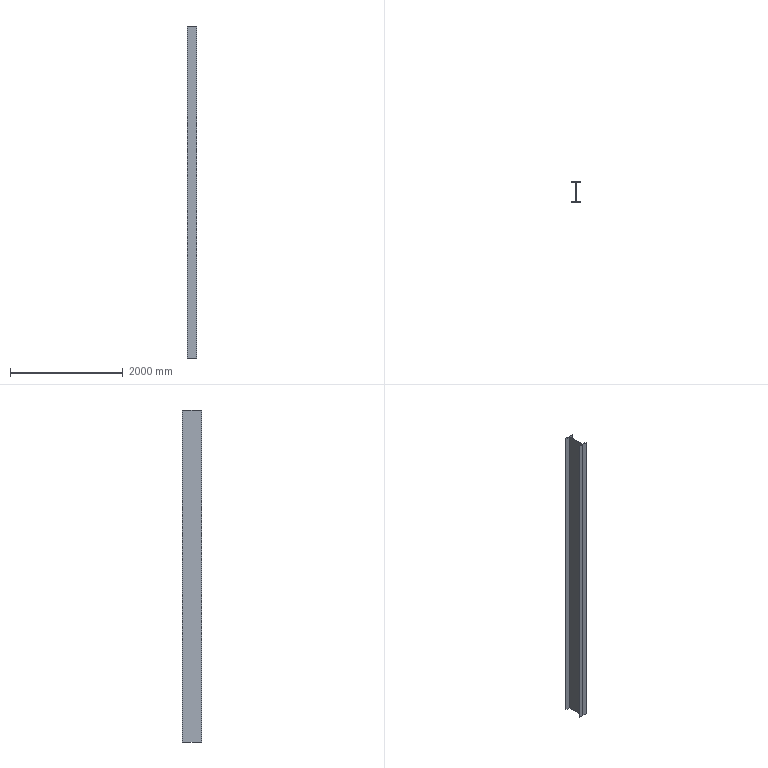Component | NX | ZHIJIA2 | 1 solid | 14 faces | box 175 x 350 x 5883 mm | volume 40004400 mm3 | plane 14
STEP:
#1=CARTESIAN_POINT('',(0.,0.,0.));
#2=DIRECTION('',(0.,0.,1.));
#3=DIRECTION('',(1.,0.,0.));
#4=AXIS2_PLACEMENT_3D('',#1,#2,#3);
#5=CARTESIAN_POINT('',(2412.5,2635.,801.349));
#6=VERTEX_POINT('',#5);
#7=CARTESIAN_POINT('',(2412.5,2625.,801.349));
#8=VERTEX_POINT('',#7);
#9=CARTESIAN_POINT('',(2412.5,2635.,801.349));
#10=DIRECTION('',(-0.,-1.,0.));
#11=VECTOR('',#10,1.);
#12=LINE('',#9,#11);
#13=CARTESIAN_POINT('',(2412.5,2635.,6684.349));
#14=DIRECTION('',(1.,-0.,0.));
#15=DIRECTION('',(0.,1.,0.));
#16=AXIS2_PLACEMENT_3D('',#13,#14,#15);
#17=PLANE('',#16);
#18=CARTESIAN_POINT('',(0.,-5883.));
#19=DIRECTION('',(-1.,0.));
#20=VECTOR('',#19,1.);
#21=LINE('',#18,#20);
#22=(GEOMETRIC_REPRESENTATION_CONTEXT(2)PARAMETRIC_REPRESENTATION_CONTEXT()REPRESENTATION_CONTEXT('',''));
#23=DEFINITIONAL_REPRESENTATION('',(#21),#22);
#24=PCURVE('',#17,#23);
#25=CARTESIAN_POINT('',(2412.5,2625.,801.349));
#26=DIRECTION('',(0.,0.,1.));
#27=DIRECTION('',(1.,0.,0.));
#28=AXIS2_PLACEMENT_3D('',#25,#26,#27);
#29=PLANE('',#28);
#30=CARTESIAN_POINT('',(0.,10.));
#31=DIRECTION('',(-0.,-1.));
#32=VECTOR('',#31,1.);
#33=LINE('',#30,#32);
#34=(GEOMETRIC_REPRESENTATION_CONTEXT(2)PARAMETRIC_REPRESENTATION_CONTEXT()REPRESENTATION_CONTEXT('',''));
#35=DEFINITIONAL_REPRESENTATION('',(#33),#34);
#36=PCURVE('',#29,#35);
#37=SURFACE_CURVE('',#12,(#24,#36),.PCURVE_S1.);
#38=EDGE_CURVE('',#6,#8,#37,.T.);
#39=ORIENTED_EDGE('',*,*,#38,.T.);
#40=CARTESIAN_POINT('',(2412.5,2625.,6684.349));
#41=VERTEX_POINT('',#40);
#42=CARTESIAN_POINT('',(2412.5,2625.,6684.349));
#43=DIRECTION('',(0.,0.,-1.));
#44=VECTOR('',#43,1.);
#45=LINE('',#42,#44);
#46=CARTESIAN_POINT('',(-10.,0.));
#47=DIRECTION('',(0.,-1.));
#48=VECTOR('',#47,1.);
#49=LINE('',#46,#48);
#50=(GEOMETRIC_REPRESENTATION_CONTEXT(2)PARAMETRIC_REPRESENTATION_CONTEXT()REPRESENTATION_CONTEXT('',''));
#51=DEFINITIONAL_REPRESENTATION('',(#49),#50);
#52=PCURVE('',#17,#51);
#53=CARTESIAN_POINT('',(2412.5,2625.,6684.349));
#54=DIRECTION('',(0.,1.,0.));
#55=DIRECTION('',(0.,0.,1.));
#56=AXIS2_PLACEMENT_3D('',#53,#54,#55);
#57=PLANE('',#56);
#58=CARTESIAN_POINT('',(0.,0.));
#59=DIRECTION('',(-1.,0.));
#60=VECTOR('',#59,1.);
#61=LINE('',#58,#60);
#62=(GEOMETRIC_REPRESENTATION_CONTEXT(2)PARAMETRIC_REPRESENTATION_CONTEXT()REPRESENTATION_CONTEXT('',''));
#63=DEFINITIONAL_REPRESENTATION('',(#61),#62);
#64=PCURVE('',#57,#63);
#65=SURFACE_CURVE('',#45,(#52,#64),.PCURVE_S1.);
#66=EDGE_CURVE('',#41,#8,#65,.T.);
#67=ORIENTED_EDGE('',*,*,#66,.F.);
#68=CARTESIAN_POINT('',(2412.5,2635.,6684.349));
#69=VERTEX_POINT('',#68);
#70=CARTESIAN_POINT('',(2412.5,2635.,6684.349));
#71=DIRECTION('',(-0.,-1.,0.));
#72=VECTOR('',#71,1.);
#73=LINE('',#70,#72);
#74=CARTESIAN_POINT('',(0.,0.));
#75=DIRECTION('',(-1.,0.));
#76=VECTOR('',#75,1.);
#77=LINE('',#74,#76);
#78=(GEOMETRIC_REPRESENTATION_CONTEXT(2)PARAMETRIC_REPRESENTATION_CONTEXT()REPRESENTATION_CONTEXT('',''));
#79=DEFINITIONAL_REPRESENTATION('',(#77),#78);
#80=PCURVE('',#17,#79);
#81=CARTESIAN_POINT('',(2412.5,2625.,6684.349));
#82=DIRECTION('',(0.,0.,1.));
#83=DIRECTION('',(1.,0.,0.));
#84=AXIS2_PLACEMENT_3D('',#81,#82,#83);
#85=PLANE('',#84);
#86=CARTESIAN_POINT('',(0.,10.));
#87=DIRECTION('',(-0.,-1.));
#88=VECTOR('',#87,1.);
#89=LINE('',#86,#88);
#90=(GEOMETRIC_REPRESENTATION_CONTEXT(2)PARAMETRIC_REPRESENTATION_CONTEXT()REPRESENTATION_CONTEXT('',''));
#91=DEFINITIONAL_REPRESENTATION('',(#89),#90);
#92=PCURVE('',#85,#91);
#93=SURFACE_CURVE('',#73,(#80,#92),.PCURVE_S1.);
#94=EDGE_CURVE('',#69,#41,#93,.T.);
#95=ORIENTED_EDGE('',*,*,#94,.F.);
#96=CARTESIAN_POINT('',(2412.5,2635.,6684.349));
#97=DIRECTION('',(0.,0.,-1.));
#98=VECTOR('',#97,1.);
#99=LINE('',#96,#98);
#100=CARTESIAN_POINT('',(0.,0.));
#101=DIRECTION('',(0.,-1.));
#102=VECTOR('',#101,1.);
#103=LINE('',#100,#102);
#104=(GEOMETRIC_REPRESENTATION_CONTEXT(2)PARAMETRIC_REPRESENTATION_CONTEXT()REPRESENTATION_CONTEXT('',''));
#105=DEFINITIONAL_REPRESENTATION('',(#103),#104);
#106=PCURVE('',#17,#105);
#107=CARTESIAN_POINT('',(2495.,2635.,6684.349));
#108=DIRECTION('',(0.,-1.,0.));
#109=DIRECTION('',(0.,0.,-1.));
#110=AXIS2_PLACEMENT_3D('',#107,#108,#109);
#111=PLANE('',#110);
#112=CARTESIAN_POINT('',(0.,-82.5));
#113=DIRECTION('',(1.,0.));
#114=VECTOR('',#113,1.);
#115=LINE('',#112,#114);
#116=(GEOMETRIC_REPRESENTATION_CONTEXT(2)PARAMETRIC_REPRESENTATION_CONTEXT()REPRESENTATION_CONTEXT('',''));
#117=DEFINITIONAL_REPRESENTATION('',(#115),#116);
#118=PCURVE('',#111,#117);
#119=SURFACE_CURVE('',#99,(#106,#118),.PCURVE_S1.);
#120=EDGE_CURVE('',#69,#6,#119,.T.);
#121=ORIENTED_EDGE('',*,*,#120,.T.);
#122=EDGE_LOOP('',(#39,#67,#95,#121));
#123=FACE_BOUND('',#122,.T.);
#124=ADVANCED_FACE('',(#123),#17,.F.);
#125=CARTESIAN_POINT('',(2587.5,2625.,801.349));
#126=VERTEX_POINT('',#125);
#127=CARTESIAN_POINT('',(2412.5,2625.,801.349));
#128=DIRECTION('',(1.,0.,0.));
#129=VECTOR('',#128,1.);
#130=LINE('',#127,#129);
#131=CARTESIAN_POINT('',(-5883.,0.));
#132=DIRECTION('',(0.,1.));
#133=VECTOR('',#132,1.);
#134=LINE('',#131,#133);
#135=(GEOMETRIC_REPRESENTATION_CONTEXT(2)PARAMETRIC_REPRESENTATION_CONTEXT()REPRESENTATION_CONTEXT('',''));
#136=DEFINITIONAL_REPRESENTATION('',(#134),#135);
#137=PCURVE('',#57,#136);
#138=CARTESIAN_POINT('',(0.,0.));
#139=DIRECTION('',(1.,0.));
#140=VECTOR('',#139,1.);
#141=LINE('',#138,#140);
#142=(GEOMETRIC_REPRESENTATION_CONTEXT(2)PARAMETRIC_REPRESENTATION_CONTEXT()REPRESENTATION_CONTEXT('',''));
#143=DEFINITIONAL_REPRESENTATION('',(#141),#142);
#144=PCURVE('',#29,#143);
#145=SURFACE_CURVE('',#130,(#137,#144),.PCURVE_S1.);
#146=EDGE_CURVE('',#8,#126,#145,.T.);
#147=ORIENTED_EDGE('',*,*,#146,.T.);
#148=CARTESIAN_POINT('',(2587.5,2625.,6684.349));
#149=VERTEX_POINT('',#148);
#150=CARTESIAN_POINT('',(2587.5,2625.,6684.349));
#151=DIRECTION('',(0.,0.,-1.));
#152=VECTOR('',#151,1.);
#153=LINE('',#150,#152);
#154=CARTESIAN_POINT('',(0.,175.));
#155=DIRECTION('',(-1.,0.));
#156=VECTOR('',#155,1.);
#157=LINE('',#154,#156);
#158=(GEOMETRIC_REPRESENTATION_CONTEXT(2)PARAMETRIC_REPRESENTATION_CONTEXT()REPRESENTATION_CONTEXT('',''));
#159=DEFINITIONAL_REPRESENTATION('',(#157),#158);
#160=PCURVE('',#57,#159);
#161=CARTESIAN_POINT('',(2587.5,2625.,6684.349));
#162=DIRECTION('',(-1.,0.,0.));
#163=DIRECTION('',(-0.,-1.,0.));
#164=AXIS2_PLACEMENT_3D('',#161,#162,#163);
#165=PLANE('',#164);
#166=CARTESIAN_POINT('',(0.,0.));
#167=DIRECTION('',(0.,-1.));
#168=VECTOR('',#167,1.);
#169=LINE('',#166,#168);
#170=(GEOMETRIC_REPRESENTATION_CONTEXT(2)PARAMETRIC_REPRESENTATION_CONTEXT()REPRESENTATION_CONTEXT('',''));
#171=DEFINITIONAL_REPRESENTATION('',(#169),#170);
#172=PCURVE('',#165,#171);
#173=SURFACE_CURVE('',#153,(#160,#172),.PCURVE_S1.);
#174=EDGE_CURVE('',#149,#126,#173,.T.);
#175=ORIENTED_EDGE('',*,*,#174,.F.);
#176=CARTESIAN_POINT('',(2412.5,2625.,6684.349));
#177=DIRECTION('',(1.,0.,0.));
#178=VECTOR('',#177,1.);
#179=LINE('',#176,#178);
#180=CARTESIAN_POINT('',(0.,0.));
#181=DIRECTION('',(0.,1.));
#182=VECTOR('',#181,1.);
#183=LINE('',#180,#182);
#184=(GEOMETRIC_REPRESENTATION_CONTEXT(2)PARAMETRIC_REPRESENTATION_CONTEXT()REPRESENTATION_CONTEXT('',''));
#185=DEFINITIONAL_REPRESENTATION('',(#183),#184);
#186=PCURVE('',#57,#185);
#187=CARTESIAN_POINT('',(0.,0.));
#188=DIRECTION('',(1.,0.));
#189=VECTOR('',#188,1.);
#190=LINE('',#187,#189);
#191=(GEOMETRIC_REPRESENTATION_CONTEXT(2)PARAMETRIC_REPRESENTATION_CONTEXT()REPRESENTATION_CONTEXT('',''));
#192=DEFINITIONAL_REPRESENTATION('',(#190),#191);
#193=PCURVE('',#85,#192);
#194=SURFACE_CURVE('',#179,(#186,#193),.PCURVE_S1.);
#195=EDGE_CURVE('',#41,#149,#194,.T.);
#196=ORIENTED_EDGE('',*,*,#195,.F.);
#197=ORIENTED_EDGE('',*,*,#66,.T.);
#198=EDGE_LOOP('',(#147,#175,#196,#197));
#199=FACE_BOUND('',#198,.T.);
#200=ADVANCED_FACE('',(#199),#57,.F.);
#201=CARTESIAN_POINT('',(2587.5,2635.,801.349));
#202=VERTEX_POINT('',#201);
#203=CARTESIAN_POINT('',(2587.5,2625.,801.349));
#204=DIRECTION('',(0.,1.,0.));
#205=VECTOR('',#204,1.);
#206=LINE('',#203,#205);
#207=CARTESIAN_POINT('',(0.,-5883.));
#208=DIRECTION('',(-1.,0.));
#209=VECTOR('',#208,1.);
#210=LINE('',#207,#209);
#211=(GEOMETRIC_REPRESENTATION_CONTEXT(2)PARAMETRIC_REPRESENTATION_CONTEXT()REPRESENTATION_CONTEXT('',''));
#212=DEFINITIONAL_REPRESENTATION('',(#210),#211);
#213=PCURVE('',#165,#212);
#214=CARTESIAN_POINT('',(175.,0.));
#215=DIRECTION('',(0.,1.));
#216=VECTOR('',#215,1.);
#217=LINE('',#214,#216);
#218=(GEOMETRIC_REPRESENTATION_CONTEXT(2)PARAMETRIC_REPRESENTATION_CONTEXT()REPRESENTATION_CONTEXT('',''));
#219=DEFINITIONAL_REPRESENTATION('',(#217),#218);
#220=PCURVE('',#29,#219);
#221=SURFACE_CURVE('',#206,(#213,#220),.PCURVE_S1.);
#222=EDGE_CURVE('',#126,#202,#221,.T.);
#223=ORIENTED_EDGE('',*,*,#222,.T.);
#224=CARTESIAN_POINT('',(2587.5,2635.,6684.349));
#225=VERTEX_POINT('',#224);
#226=CARTESIAN_POINT('',(2587.5,2635.,6684.349));
#227=DIRECTION('',(0.,0.,-1.));
#228=VECTOR('',#227,1.);
#229=LINE('',#226,#228);
#230=CARTESIAN_POINT('',(-10.,0.));
#231=DIRECTION('',(0.,-1.));
#232=VECTOR('',#231,1.);
#233=LINE('',#230,#232);
#234=(GEOMETRIC_REPRESENTATION_CONTEXT(2)PARAMETRIC_REPRESENTATION_CONTEXT()REPRESENTATION_CONTEXT('',''));
#235=DEFINITIONAL_REPRESENTATION('',(#233),#234);
#236=PCURVE('',#165,#235);
#237=CARTESIAN_POINT('',(2587.5,2635.,6684.349));
#238=DIRECTION('',(0.,-1.,0.));
#239=DIRECTION('',(0.,0.,-1.));
#240=AXIS2_PLACEMENT_3D('',#237,#238,#239);
#241=PLANE('',#240);
#242=CARTESIAN_POINT('',(0.,0.));
#243=DIRECTION('',(1.,0.));
#244=VECTOR('',#243,1.);
#245=LINE('',#242,#244);
#246=(GEOMETRIC_REPRESENTATION_CONTEXT(2)PARAMETRIC_REPRESENTATION_CONTEXT()REPRESENTATION_CONTEXT('',''));
#247=DEFINITIONAL_REPRESENTATION('',(#245),#246);
#248=PCURVE('',#241,#247);
#249=SURFACE_CURVE('',#229,(#236,#248),.PCURVE_S1.);
#250=EDGE_CURVE('',#225,#202,#249,.T.);
#251=ORIENTED_EDGE('',*,*,#250,.F.);
#252=CARTESIAN_POINT('',(2587.5,2625.,6684.349));
#253=DIRECTION('',(0.,1.,0.));
#254=VECTOR('',#253,1.);
#255=LINE('',#252,#254);
#256=CARTESIAN_POINT('',(0.,0.));
#257=DIRECTION('',(-1.,0.));
#258=VECTOR('',#257,1.);
#259=LINE('',#256,#258);
#260=(GEOMETRIC_REPRESENTATION_CONTEXT(2)PARAMETRIC_REPRESENTATION_CONTEXT()REPRESENTATION_CONTEXT('',''));
#261=DEFINITIONAL_REPRESENTATION('',(#259),#260);
#262=PCURVE('',#165,#261);
#263=CARTESIAN_POINT('',(175.,0.));
#264=DIRECTION('',(0.,1.));
#265=VECTOR('',#264,1.);
#266=LINE('',#263,#265);
#267=(GEOMETRIC_REPRESENTATION_CONTEXT(2)PARAMETRIC_REPRESENTATION_CONTEXT()REPRESENTATION_CONTEXT('',''));
#268=DEFINITIONAL_REPRESENTATION('',(#266),#267);
#269=PCURVE('',#85,#268);
#270=SURFACE_CURVE('',#255,(#262,#269),.PCURVE_S1.);
#271=EDGE_CURVE('',#149,#225,#270,.T.);
#272=ORIENTED_EDGE('',*,*,#271,.F.);
#273=ORIENTED_EDGE('',*,*,#174,.T.);
#274=EDGE_LOOP('',(#223,#251,#272,#273));
#275=FACE_BOUND('',#274,.T.);
#276=ADVANCED_FACE('',(#275),#165,.F.);
#277=CARTESIAN_POINT('',(2505.,2635.,801.349));
#278=VERTEX_POINT('',#277);
#279=CARTESIAN_POINT('',(2587.5,2635.,801.349));
#280=DIRECTION('',(-1.,0.,0.));
#281=VECTOR('',#280,1.);
#282=LINE('',#279,#281);
#283=CARTESIAN_POINT('',(5883.,0.));
#284=DIRECTION('',(0.,-1.));
#285=VECTOR('',#284,1.);
#286=LINE('',#283,#285);
#287=(GEOMETRIC_REPRESENTATION_CONTEXT(2)PARAMETRIC_REPRESENTATION_CONTEXT()REPRESENTATION_CONTEXT('',''));
#288=DEFINITIONAL_REPRESENTATION('',(#286),#287);
#289=PCURVE('',#241,#288);
#290=CARTESIAN_POINT('',(175.,10.));
#291=DIRECTION('',(-1.,0.));
#292=VECTOR('',#291,1.);
#293=LINE('',#290,#292);
#294=(GEOMETRIC_REPRESENTATION_CONTEXT(2)PARAMETRIC_REPRESENTATION_CONTEXT()REPRESENTATION_CONTEXT('',''));
#295=DEFINITIONAL_REPRESENTATION('',(#293),#294);
#296=PCURVE('',#29,#295);
#297=SURFACE_CURVE('',#282,(#289,#296),.PCURVE_S1.);
#298=EDGE_CURVE('',#202,#278,#297,.T.);
#299=ORIENTED_EDGE('',*,*,#298,.T.);
#300=CARTESIAN_POINT('',(2505.,2635.,6684.349));
#301=VERTEX_POINT('',#300);
#302=CARTESIAN_POINT('',(2505.,2635.,6684.349));
#303=DIRECTION('',(0.,0.,-1.));
#304=VECTOR('',#303,1.);
#305=LINE('',#302,#304);
#306=CARTESIAN_POINT('',(0.,-82.5));
#307=DIRECTION('',(1.,0.));
#308=VECTOR('',#307,1.);
#309=LINE('',#306,#308);
#310=(GEOMETRIC_REPRESENTATION_CONTEXT(2)PARAMETRIC_REPRESENTATION_CONTEXT()REPRESENTATION_CONTEXT('',''));
#311=DEFINITIONAL_REPRESENTATION('',(#309),#310);
#312=PCURVE('',#241,#311);
#313=CARTESIAN_POINT('',(2505.,2635.,6684.349));
#314=DIRECTION('',(-1.,0.,0.));
#315=DIRECTION('',(-0.,-1.,0.));
#316=AXIS2_PLACEMENT_3D('',#313,#314,#315);
#317=PLANE('',#316);
#318=CARTESIAN_POINT('',(0.,0.));
#319=DIRECTION('',(0.,-1.));
#320=VECTOR('',#319,1.);
#321=LINE('',#318,#320);
#322=(GEOMETRIC_REPRESENTATION_CONTEXT(2)PARAMETRIC_REPRESENTATION_CONTEXT()REPRESENTATION_CONTEXT('',''));
#323=DEFINITIONAL_REPRESENTATION('',(#321),#322);
#324=PCURVE('',#317,#323);
#325=SURFACE_CURVE('',#305,(#312,#324),.PCURVE_S1.);
#326=EDGE_CURVE('',#301,#278,#325,.T.);
#327=ORIENTED_EDGE('',*,*,#326,.F.);
#328=CARTESIAN_POINT('',(2587.5,2635.,6684.349));
#329=DIRECTION('',(-1.,0.,0.));
#330=VECTOR('',#329,1.);
#331=LINE('',#328,#330);
#332=CARTESIAN_POINT('',(0.,0.));
#333=DIRECTION('',(0.,-1.));
#334=VECTOR('',#333,1.);
#335=LINE('',#332,#334);
#336=(GEOMETRIC_REPRESENTATION_CONTEXT(2)PARAMETRIC_REPRESENTATION_CONTEXT()REPRESENTATION_CONTEXT('',''));
#337=DEFINITIONAL_REPRESENTATION('',(#335),#336);
#338=PCURVE('',#241,#337);
#339=CARTESIAN_POINT('',(175.,10.));
#340=DIRECTION('',(-1.,0.));
#341=VECTOR('',#340,1.);
#342=LINE('',#339,#341);
#343=(GEOMETRIC_REPRESENTATION_CONTEXT(2)PARAMETRIC_REPRESENTATION_CONTEXT()REPRESENTATION_CONTEXT('',''));
#344=DEFINITIONAL_REPRESENTATION('',(#342),#343);
#345=PCURVE('',#85,#344);
#346=SURFACE_CURVE('',#331,(#338,#345),.PCURVE_S1.);
#347=EDGE_CURVE('',#225,#301,#346,.T.);
#348=ORIENTED_EDGE('',*,*,#347,.F.);
#349=ORIENTED_EDGE('',*,*,#250,.T.);
#350=EDGE_LOOP('',(#299,#327,#348,#349));
#351=FACE_BOUND('',#350,.T.);
#352=ADVANCED_FACE('',(#351),#241,.F.);
#353=CARTESIAN_POINT('',(2505.,2965.,801.349));
#354=VERTEX_POINT('',#353);
#355=CARTESIAN_POINT('',(2505.,2635.,801.349));
#356=DIRECTION('',(0.,1.,0.));
#357=VECTOR('',#356,1.);
#358=LINE('',#355,#357);
#359=CARTESIAN_POINT('',(0.,-5883.));
#360=DIRECTION('',(-1.,0.));
#361=VECTOR('',#360,1.);
#362=LINE('',#359,#361);
#363=(GEOMETRIC_REPRESENTATION_CONTEXT(2)PARAMETRIC_REPRESENTATION_CONTEXT()REPRESENTATION_CONTEXT('',''));
#364=DEFINITIONAL_REPRESENTATION('',(#362),#363);
#365=PCURVE('',#317,#364);
#366=CARTESIAN_POINT('',(92.5,10.));
#367=DIRECTION('',(0.,1.));
#368=VECTOR('',#367,1.);
#369=LINE('',#366,#368);
#370=(GEOMETRIC_REPRESENTATION_CONTEXT(2)PARAMETRIC_REPRESENTATION_CONTEXT()REPRESENTATION_CONTEXT('',''));
#371=DEFINITIONAL_REPRESENTATION('',(#369),#370);
#372=PCURVE('',#29,#371);
#373=SURFACE_CURVE('',#358,(#365,#372),.PCURVE_S1.);
#374=EDGE_CURVE('',#278,#354,#373,.T.);
#375=ORIENTED_EDGE('',*,*,#374,.T.);
#376=CARTESIAN_POINT('',(2505.,2965.,6684.349));
#377=VERTEX_POINT('',#376);
#378=CARTESIAN_POINT('',(2505.,2965.,6684.349));
#379=DIRECTION('',(0.,0.,-1.));
#380=VECTOR('',#379,1.);
#381=LINE('',#378,#380);
#382=CARTESIAN_POINT('',(-330.,0.));
#383=DIRECTION('',(0.,-1.));
#384=VECTOR('',#383,1.);
#385=LINE('',#382,#384);
#386=(GEOMETRIC_REPRESENTATION_CONTEXT(2)PARAMETRIC_REPRESENTATION_CONTEXT()REPRESENTATION_CONTEXT('',''));
#387=DEFINITIONAL_REPRESENTATION('',(#385),#386);
#388=PCURVE('',#317,#387);
#389=CARTESIAN_POINT('',(2505.,2965.,6684.349));
#390=DIRECTION('',(0.,1.,0.));
#391=DIRECTION('',(0.,0.,1.));
#392=AXIS2_PLACEMENT_3D('',#389,#390,#391);
#393=PLANE('',#392);
#394=CARTESIAN_POINT('',(0.,0.));
#395=DIRECTION('',(-1.,0.));
#396=VECTOR('',#395,1.);
#397=LINE('',#394,#396);
#398=(GEOMETRIC_REPRESENTATION_CONTEXT(2)PARAMETRIC_REPRESENTATION_CONTEXT()REPRESENTATION_CONTEXT('',''));
#399=DEFINITIONAL_REPRESENTATION('',(#397),#398);
#400=PCURVE('',#393,#399);
#401=SURFACE_CURVE('',#381,(#388,#400),.PCURVE_S1.);
#402=EDGE_CURVE('',#377,#354,#401,.T.);
#403=ORIENTED_EDGE('',*,*,#402,.F.);
#404=CARTESIAN_POINT('',(2505.,2635.,6684.349));
#405=DIRECTION('',(0.,1.,0.));
#406=VECTOR('',#405,1.);
#407=LINE('',#404,#406);
#408=CARTESIAN_POINT('',(0.,0.));
#409=DIRECTION('',(-1.,0.));
#410=VECTOR('',#409,1.);
#411=LINE('',#408,#410);
#412=(GEOMETRIC_REPRESENTATION_CONTEXT(2)PARAMETRIC_REPRESENTATION_CONTEXT()REPRESENTATION_CONTEXT('',''));
#413=DEFINITIONAL_REPRESENTATION('',(#411),#412);
#414=PCURVE('',#317,#413);
#415=CARTESIAN_POINT('',(92.5,10.));
#416=DIRECTION('',(0.,1.));
#417=VECTOR('',#416,1.);
#418=LINE('',#415,#417);
#419=(GEOMETRIC_REPRESENTATION_CONTEXT(2)PARAMETRIC_REPRESENTATION_CONTEXT()REPRESENTATION_CONTEXT('',''));
#420=DEFINITIONAL_REPRESENTATION('',(#418),#419);
#421=PCURVE('',#85,#420);
#422=SURFACE_CURVE('',#407,(#414,#421),.PCURVE_S1.);
#423=EDGE_CURVE('',#301,#377,#422,.T.);
#424=ORIENTED_EDGE('',*,*,#423,.F.);
#425=ORIENTED_EDGE('',*,*,#326,.T.);
#426=EDGE_LOOP('',(#375,#403,#424,#425));
#427=FACE_BOUND('',#426,.T.);
#428=ADVANCED_FACE('',(#427),#317,.F.);
#429=CARTESIAN_POINT('',(2587.5,2965.,801.349));
#430=VERTEX_POINT('',#429);
#431=CARTESIAN_POINT('',(2505.,2965.,801.349));
#432=DIRECTION('',(1.,0.,0.));
#433=VECTOR('',#432,1.);
#434=LINE('',#431,#433);
#435=CARTESIAN_POINT('',(-5883.,0.));
#436=DIRECTION('',(0.,1.));
#437=VECTOR('',#436,1.);
#438=LINE('',#435,#437);
#439=(GEOMETRIC_REPRESENTATION_CONTEXT(2)PARAMETRIC_REPRESENTATION_CONTEXT()REPRESENTATION_CONTEXT('',''));
#440=DEFINITIONAL_REPRESENTATION('',(#438),#439);
#441=PCURVE('',#393,#440);
#442=CARTESIAN_POINT('',(92.5,340.));
#443=DIRECTION('',(1.,0.));
#444=VECTOR('',#443,1.);
#445=LINE('',#442,#444);
#446=(GEOMETRIC_REPRESENTATION_CONTEXT(2)PARAMETRIC_REPRESENTATION_CONTEXT()REPRESENTATION_CONTEXT('',''));
#447=DEFINITIONAL_REPRESENTATION('',(#445),#446);
#448=PCURVE('',#29,#447);
#449=SURFACE_CURVE('',#434,(#441,#448),.PCURVE_S1.);
#450=EDGE_CURVE('',#354,#430,#449,.T.);
#451=ORIENTED_EDGE('',*,*,#450,.T.);
#452=CARTESIAN_POINT('',(2587.5,2965.,6684.349));
#453=VERTEX_POINT('',#452);
#454=CARTESIAN_POINT('',(2587.5,2965.,6684.349));
#455=DIRECTION('',(0.,0.,-1.));
#456=VECTOR('',#455,1.);
#457=LINE('',#454,#456);
#458=CARTESIAN_POINT('',(0.,82.5));
#459=DIRECTION('',(-1.,0.));
#460=VECTOR('',#459,1.);
#461=LINE('',#458,#460);
#462=(GEOMETRIC_REPRESENTATION_CONTEXT(2)PARAMETRIC_REPRESENTATION_CONTEXT()REPRESENTATION_CONTEXT('',''));
#463=DEFINITIONAL_REPRESENTATION('',(#461),#462);
#464=PCURVE('',#393,#463);
#465=CARTESIAN_POINT('',(2587.5,2965.,6684.349));
#466=DIRECTION('',(-1.,0.,0.));
#467=DIRECTION('',(-0.,-1.,0.));
#468=AXIS2_PLACEMENT_3D('',#465,#466,#467);
#469=PLANE('',#468);
#470=CARTESIAN_POINT('',(0.,0.));
#471=DIRECTION('',(0.,-1.));
#472=VECTOR('',#471,1.);
#473=LINE('',#470,#472);
#474=(GEOMETRIC_REPRESENTATION_CONTEXT(2)PARAMETRIC_REPRESENTATION_CONTEXT()REPRESENTATION_CONTEXT('',''));
#475=DEFINITIONAL_REPRESENTATION('',(#473),#474);
#476=PCURVE('',#469,#475);
#477=SURFACE_CURVE('',#457,(#464,#476),.PCURVE_S1.);
#478=EDGE_CURVE('',#453,#430,#477,.T.);
#479=ORIENTED_EDGE('',*,*,#478,.F.);
#480=CARTESIAN_POINT('',(2505.,2965.,6684.349));
#481=DIRECTION('',(1.,0.,0.));
#482=VECTOR('',#481,1.);
#483=LINE('',#480,#482);
#484=CARTESIAN_POINT('',(0.,0.));
#485=DIRECTION('',(0.,1.));
#486=VECTOR('',#485,1.);
#487=LINE('',#484,#486);
#488=(GEOMETRIC_REPRESENTATION_CONTEXT(2)PARAMETRIC_REPRESENTATION_CONTEXT()REPRESENTATION_CONTEXT('',''));
#489=DEFINITIONAL_REPRESENTATION('',(#487),#488);
#490=PCURVE('',#393,#489);
#491=CARTESIAN_POINT('',(92.5,340.));
#492=DIRECTION('',(1.,0.));
#493=VECTOR('',#492,1.);
#494=LINE('',#491,#493);
#495=(GEOMETRIC_REPRESENTATION_CONTEXT(2)PARAMETRIC_REPRESENTATION_CONTEXT()REPRESENTATION_CONTEXT('',''));
#496=DEFINITIONAL_REPRESENTATION('',(#494),#495);
#497=PCURVE('',#85,#496);
#498=SURFACE_CURVE('',#483,(#490,#497),.PCURVE_S1.);
#499=EDGE_CURVE('',#377,#453,#498,.T.);
#500=ORIENTED_EDGE('',*,*,#499,.F.);
#501=ORIENTED_EDGE('',*,*,#402,.T.);
#502=EDGE_LOOP('',(#451,#479,#500,#501));
#503=FACE_BOUND('',#502,.T.);
#504=ADVANCED_FACE('',(#503),#393,.F.);
#505=CARTESIAN_POINT('',(2587.5,2975.,801.349));
#506=VERTEX_POINT('',#505);
#507=CARTESIAN_POINT('',(2587.5,2965.,801.349));
#508=DIRECTION('',(0.,1.,0.));
#509=VECTOR('',#508,1.);
#510=LINE('',#507,#509);
#511=CARTESIAN_POINT('',(0.,-5883.));
#512=DIRECTION('',(-1.,0.));
#513=VECTOR('',#512,1.);
#514=LINE('',#511,#513);
#515=(GEOMETRIC_REPRESENTATION_CONTEXT(2)PARAMETRIC_REPRESENTATION_CONTEXT()REPRESENTATION_CONTEXT('',''));
#516=DEFINITIONAL_REPRESENTATION('',(#514),#515);
#517=PCURVE('',#469,#516);
#518=CARTESIAN_POINT('',(175.,340.));
#519=DIRECTION('',(0.,1.));
#520=VECTOR('',#519,1.);
#521=LINE('',#518,#520);
#522=(GEOMETRIC_REPRESENTATION_CONTEXT(2)PARAMETRIC_REPRESENTATION_CONTEXT()REPRESENTATION_CONTEXT('',''));
#523=DEFINITIONAL_REPRESENTATION('',(#521),#522);
#524=PCURVE('',#29,#523);
#525=SURFACE_CURVE('',#510,(#517,#524),.PCURVE_S1.);
#526=EDGE_CURVE('',#430,#506,#525,.T.);
#527=ORIENTED_EDGE('',*,*,#526,.T.);
#528=CARTESIAN_POINT('',(2587.5,2975.,6684.349));
#529=VERTEX_POINT('',#528);
#530=CARTESIAN_POINT('',(2587.5,2975.,6684.349));
#531=DIRECTION('',(0.,0.,-1.));
#532=VECTOR('',#531,1.);
#533=LINE('',#530,#532);
#534=CARTESIAN_POINT('',(-10.,0.));
#535=DIRECTION('',(0.,-1.));
#536=VECTOR('',#535,1.);
#537=LINE('',#534,#536);
#538=(GEOMETRIC_REPRESENTATION_CONTEXT(2)PARAMETRIC_REPRESENTATION_CONTEXT()REPRESENTATION_CONTEXT('',''));
#539=DEFINITIONAL_REPRESENTATION('',(#537),#538);
#540=PCURVE('',#469,#539);
#541=CARTESIAN_POINT('',(2587.5,2975.,6684.349));
#542=DIRECTION('',(0.,-1.,0.));
#543=DIRECTION('',(0.,0.,-1.));
#544=AXIS2_PLACEMENT_3D('',#541,#542,#543);
#545=PLANE('',#544);
#546=CARTESIAN_POINT('',(0.,0.));
#547=DIRECTION('',(1.,0.));
#548=VECTOR('',#547,1.);
#549=LINE('',#546,#548);
#550=(GEOMETRIC_REPRESENTATION_CONTEXT(2)PARAMETRIC_REPRESENTATION_CONTEXT()REPRESENTATION_CONTEXT('',''));
#551=DEFINITIONAL_REPRESENTATION('',(#549),#550);
#552=PCURVE('',#545,#551);
#553=SURFACE_CURVE('',#533,(#540,#552),.PCURVE_S1.);
#554=EDGE_CURVE('',#529,#506,#553,.T.);
#555=ORIENTED_EDGE('',*,*,#554,.F.);
#556=CARTESIAN_POINT('',(2587.5,2965.,6684.349));
#557=DIRECTION('',(0.,1.,0.));
#558=VECTOR('',#557,1.);
#559=LINE('',#556,#558);
#560=CARTESIAN_POINT('',(0.,0.));
#561=DIRECTION('',(-1.,0.));
#562=VECTOR('',#561,1.);
#563=LINE('',#560,#562);
#564=(GEOMETRIC_REPRESENTATION_CONTEXT(2)PARAMETRIC_REPRESENTATION_CONTEXT()REPRESENTATION_CONTEXT('',''));
#565=DEFINITIONAL_REPRESENTATION('',(#563),#564);
#566=PCURVE('',#469,#565);
#567=CARTESIAN_POINT('',(175.,340.));
#568=DIRECTION('',(0.,1.));
#569=VECTOR('',#568,1.);
#570=LINE('',#567,#569);
#571=(GEOMETRIC_REPRESENTATION_CONTEXT(2)PARAMETRIC_REPRESENTATION_CONTEXT()REPRESENTATION_CONTEXT('',''));
#572=DEFINITIONAL_REPRESENTATION('',(#570),#571);
#573=PCURVE('',#85,#572);
#574=SURFACE_CURVE('',#559,(#566,#573),.PCURVE_S1.);
#575=EDGE_CURVE('',#453,#529,#574,.T.);
#576=ORIENTED_EDGE('',*,*,#575,.F.);
#577=ORIENTED_EDGE('',*,*,#478,.T.);
#578=EDGE_LOOP('',(#527,#555,#576,#577));
#579=FACE_BOUND('',#578,.T.);
#580=ADVANCED_FACE('',(#579),#469,.F.);
#581=CARTESIAN_POINT('',(2412.5,2975.,801.349));
#582=VERTEX_POINT('',#581);
#583=CARTESIAN_POINT('',(2587.5,2975.,801.349));
#584=DIRECTION('',(-1.,0.,0.));
#585=VECTOR('',#584,1.);
#586=LINE('',#583,#585);
#587=CARTESIAN_POINT('',(5883.,0.));
#588=DIRECTION('',(0.,-1.));
#589=VECTOR('',#588,1.);
#590=LINE('',#587,#589);
#591=(GEOMETRIC_REPRESENTATION_CONTEXT(2)PARAMETRIC_REPRESENTATION_CONTEXT()REPRESENTATION_CONTEXT('',''));
#592=DEFINITIONAL_REPRESENTATION('',(#590),#591);
#593=PCURVE('',#545,#592);
#594=CARTESIAN_POINT('',(175.,350.));
#595=DIRECTION('',(-1.,0.));
#596=VECTOR('',#595,1.);
#597=LINE('',#594,#596);
#598=(GEOMETRIC_REPRESENTATION_CONTEXT(2)PARAMETRIC_REPRESENTATION_CONTEXT()REPRESENTATION_CONTEXT('',''));
#599=DEFINITIONAL_REPRESENTATION('',(#597),#598);
#600=PCURVE('',#29,#599);
#601=SURFACE_CURVE('',#586,(#593,#600),.PCURVE_S1.);
#602=EDGE_CURVE('',#506,#582,#601,.T.);
#603=ORIENTED_EDGE('',*,*,#602,.T.);
#604=CARTESIAN_POINT('',(2412.5,2975.,6684.349));
#605=VERTEX_POINT('',#604);
#606=CARTESIAN_POINT('',(2412.5,2975.,6684.349));
#607=DIRECTION('',(0.,0.,-1.));
#608=VECTOR('',#607,1.);
#609=LINE('',#606,#608);
#610=CARTESIAN_POINT('',(0.,-175.));
#611=DIRECTION('',(1.,0.));
#612=VECTOR('',#611,1.);
#613=LINE('',#610,#612);
#614=(GEOMETRIC_REPRESENTATION_CONTEXT(2)PARAMETRIC_REPRESENTATION_CONTEXT()REPRESENTATION_CONTEXT('',''));
#615=DEFINITIONAL_REPRESENTATION('',(#613),#614);
#616=PCURVE('',#545,#615);
#617=CARTESIAN_POINT('',(2412.5,2975.,6684.349));
#618=DIRECTION('',(1.,-0.,0.));
#619=DIRECTION('',(0.,1.,0.));
#620=AXIS2_PLACEMENT_3D('',#617,#618,#619);
#621=PLANE('',#620);
#622=CARTESIAN_POINT('',(0.,0.));
#623=DIRECTION('',(0.,-1.));
#624=VECTOR('',#623,1.);
#625=LINE('',#622,#624);
#626=(GEOMETRIC_REPRESENTATION_CONTEXT(2)PARAMETRIC_REPRESENTATION_CONTEXT()REPRESENTATION_CONTEXT('',''));
#627=DEFINITIONAL_REPRESENTATION('',(#625),#626);
#628=PCURVE('',#621,#627);
#629=SURFACE_CURVE('',#609,(#616,#628),.PCURVE_S1.);
#630=EDGE_CURVE('',#605,#582,#629,.T.);
#631=ORIENTED_EDGE('',*,*,#630,.F.);
#632=CARTESIAN_POINT('',(2587.5,2975.,6684.349));
#633=DIRECTION('',(-1.,0.,0.));
#634=VECTOR('',#633,1.);
#635=LINE('',#632,#634);
#636=CARTESIAN_POINT('',(0.,0.));
#637=DIRECTION('',(0.,-1.));
#638=VECTOR('',#637,1.);
#639=LINE('',#636,#638);
#640=(GEOMETRIC_REPRESENTATION_CONTEXT(2)PARAMETRIC_REPRESENTATION_CONTEXT()REPRESENTATION_CONTEXT('',''));
#641=DEFINITIONAL_REPRESENTATION('',(#639),#640);
#642=PCURVE('',#545,#641);
#643=CARTESIAN_POINT('',(175.,350.));
#644=DIRECTION('',(-1.,0.));
#645=VECTOR('',#644,1.);
#646=LINE('',#643,#645);
#647=(GEOMETRIC_REPRESENTATION_CONTEXT(2)PARAMETRIC_REPRESENTATION_CONTEXT()REPRESENTATION_CONTEXT('',''));
#648=DEFINITIONAL_REPRESENTATION('',(#646),#647);
#649=PCURVE('',#85,#648);
#650=SURFACE_CURVE('',#635,(#642,#649),.PCURVE_S1.);
#651=EDGE_CURVE('',#529,#605,#650,.T.);
#652=ORIENTED_EDGE('',*,*,#651,.F.);
#653=ORIENTED_EDGE('',*,*,#554,.T.);
#654=EDGE_LOOP('',(#603,#631,#652,#653));
#655=FACE_BOUND('',#654,.T.);
#656=ADVANCED_FACE('',(#655),#545,.F.);
#657=CARTESIAN_POINT('',(2412.5,2965.,801.349));
#658=VERTEX_POINT('',#657);
#659=CARTESIAN_POINT('',(2412.5,2975.,801.349));
#660=DIRECTION('',(-0.,-1.,0.));
#661=VECTOR('',#660,1.);
#662=LINE('',#659,#661);
#663=CARTESIAN_POINT('',(0.,-5883.));
#664=DIRECTION('',(-1.,0.));
#665=VECTOR('',#664,1.);
#666=LINE('',#663,#665);
#667=(GEOMETRIC_REPRESENTATION_CONTEXT(2)PARAMETRIC_REPRESENTATION_CONTEXT()REPRESENTATION_CONTEXT('',''));
#668=DEFINITIONAL_REPRESENTATION('',(#666),#667);
#669=PCURVE('',#621,#668);
#670=CARTESIAN_POINT('',(0.,350.));
#671=DIRECTION('',(-0.,-1.));
#672=VECTOR('',#671,1.);
#673=LINE('',#670,#672);
#674=(GEOMETRIC_REPRESENTATION_CONTEXT(2)PARAMETRIC_REPRESENTATION_CONTEXT()REPRESENTATION_CONTEXT('',''));
#675=DEFINITIONAL_REPRESENTATION('',(#673),#674);
#676=PCURVE('',#29,#675);
#677=SURFACE_CURVE('',#662,(#669,#676),.PCURVE_S1.);
#678=EDGE_CURVE('',#582,#658,#677,.T.);
#679=ORIENTED_EDGE('',*,*,#678,.T.);
#680=CARTESIAN_POINT('',(2412.5,2965.,6684.349));
#681=VERTEX_POINT('',#680);
#682=CARTESIAN_POINT('',(2412.5,2965.,6684.349));
#683=DIRECTION('',(0.,0.,-1.));
#684=VECTOR('',#683,1.);
#685=LINE('',#682,#684);
#686=CARTESIAN_POINT('',(-10.,0.));
#687=DIRECTION('',(0.,-1.));
#688=VECTOR('',#687,1.);
#689=LINE('',#686,#688);
#690=(GEOMETRIC_REPRESENTATION_CONTEXT(2)PARAMETRIC_REPRESENTATION_CONTEXT()REPRESENTATION_CONTEXT('',''));
#691=DEFINITIONAL_REPRESENTATION('',(#689),#690);
#692=PCURVE('',#621,#691);
#693=CARTESIAN_POINT('',(2412.5,2965.,6684.349));
#694=DIRECTION('',(0.,1.,0.));
#695=DIRECTION('',(0.,0.,1.));
#696=AXIS2_PLACEMENT_3D('',#693,#694,#695);
#697=PLANE('',#696);
#698=CARTESIAN_POINT('',(0.,0.));
#699=DIRECTION('',(-1.,0.));
#700=VECTOR('',#699,1.);
#701=LINE('',#698,#700);
#702=(GEOMETRIC_REPRESENTATION_CONTEXT(2)PARAMETRIC_REPRESENTATION_CONTEXT()REPRESENTATION_CONTEXT('',''));
#703=DEFINITIONAL_REPRESENTATION('',(#701),#702);
#704=PCURVE('',#697,#703);
#705=SURFACE_CURVE('',#685,(#692,#704),.PCURVE_S1.);
#706=EDGE_CURVE('',#681,#658,#705,.T.);
#707=ORIENTED_EDGE('',*,*,#706,.F.);
#708=CARTESIAN_POINT('',(2412.5,2975.,6684.349));
#709=DIRECTION('',(-0.,-1.,0.));
#710=VECTOR('',#709,1.);
#711=LINE('',#708,#710);
#712=CARTESIAN_POINT('',(0.,0.));
#713=DIRECTION('',(-1.,0.));
#714=VECTOR('',#713,1.);
#715=LINE('',#712,#714);
#716=(GEOMETRIC_REPRESENTATION_CONTEXT(2)PARAMETRIC_REPRESENTATION_CONTEXT()REPRESENTATION_CONTEXT('',''));
#717=DEFINITIONAL_REPRESENTATION('',(#715),#716);
#718=PCURVE('',#621,#717);
#719=CARTESIAN_POINT('',(0.,350.));
#720=DIRECTION('',(-0.,-1.));
#721=VECTOR('',#720,1.);
#722=LINE('',#719,#721);
#723=(GEOMETRIC_REPRESENTATION_CONTEXT(2)PARAMETRIC_REPRESENTATION_CONTEXT()REPRESENTATION_CONTEXT('',''));
#724=DEFINITIONAL_REPRESENTATION('',(#722),#723);
#725=PCURVE('',#85,#724);
#726=SURFACE_CURVE('',#711,(#718,#725),.PCURVE_S1.);
#727=EDGE_CURVE('',#605,#681,#726,.T.);
#728=ORIENTED_EDGE('',*,*,#727,.F.);
#729=ORIENTED_EDGE('',*,*,#630,.T.);
#730=EDGE_LOOP('',(#679,#707,#728,#729));
#731=FACE_BOUND('',#730,.T.);
#732=ADVANCED_FACE('',(#731),#621,.F.);
#733=CARTESIAN_POINT('',(2495.,2965.,801.349));
#734=VERTEX_POINT('',#733);
#735=CARTESIAN_POINT('',(2412.5,2965.,801.349));
#736=DIRECTION('',(1.,0.,0.));
#737=VECTOR('',#736,1.);
#738=LINE('',#735,#737);
#739=CARTESIAN_POINT('',(-5883.,0.));
#740=DIRECTION('',(0.,1.));
#741=VECTOR('',#740,1.);
#742=LINE('',#739,#741);
#743=(GEOMETRIC_REPRESENTATION_CONTEXT(2)PARAMETRIC_REPRESENTATION_CONTEXT()REPRESENTATION_CONTEXT('',''));
#744=DEFINITIONAL_REPRESENTATION('',(#742),#743);
#745=PCURVE('',#697,#744);
#746=CARTESIAN_POINT('',(0.,340.));
#747=DIRECTION('',(1.,0.));
#748=VECTOR('',#747,1.);
#749=LINE('',#746,#748);
#750=(GEOMETRIC_REPRESENTATION_CONTEXT(2)PARAMETRIC_REPRESENTATION_CONTEXT()REPRESENTATION_CONTEXT('',''));
#751=DEFINITIONAL_REPRESENTATION('',(#749),#750);
#752=PCURVE('',#29,#751);
#753=SURFACE_CURVE('',#738,(#745,#752),.PCURVE_S1.);
#754=EDGE_CURVE('',#658,#734,#753,.T.);
#755=ORIENTED_EDGE('',*,*,#754,.T.);
#756=CARTESIAN_POINT('',(2495.,2965.,6684.349));
#757=VERTEX_POINT('',#756);
#758=CARTESIAN_POINT('',(2495.,2965.,6684.349));
#759=DIRECTION('',(0.,0.,-1.));
#760=VECTOR('',#759,1.);
#761=LINE('',#758,#760);
#762=CARTESIAN_POINT('',(0.,82.5));
#763=DIRECTION('',(-1.,0.));
#764=VECTOR('',#763,1.);
#765=LINE('',#762,#764);
#766=(GEOMETRIC_REPRESENTATION_CONTEXT(2)PARAMETRIC_REPRESENTATION_CONTEXT()REPRESENTATION_CONTEXT('',''));
#767=DEFINITIONAL_REPRESENTATION('',(#765),#766);
#768=PCURVE('',#697,#767);
#769=CARTESIAN_POINT('',(2495.,2965.,6684.349));
#770=DIRECTION('',(1.,-0.,0.));
#771=DIRECTION('',(0.,1.,0.));
#772=AXIS2_PLACEMENT_3D('',#769,#770,#771);
#773=PLANE('',#772);
#774=CARTESIAN_POINT('',(0.,0.));
#775=DIRECTION('',(0.,-1.));
#776=VECTOR('',#775,1.);
#777=LINE('',#774,#776);
#778=(GEOMETRIC_REPRESENTATION_CONTEXT(2)PARAMETRIC_REPRESENTATION_CONTEXT()REPRESENTATION_CONTEXT('',''));
#779=DEFINITIONAL_REPRESENTATION('',(#777),#778);
#780=PCURVE('',#773,#779);
#781=SURFACE_CURVE('',#761,(#768,#780),.PCURVE_S1.);
#782=EDGE_CURVE('',#757,#734,#781,.T.);
#783=ORIENTED_EDGE('',*,*,#782,.F.);
#784=CARTESIAN_POINT('',(2412.5,2965.,6684.349));
#785=DIRECTION('',(1.,0.,0.));
#786=VECTOR('',#785,1.);
#787=LINE('',#784,#786);
#788=CARTESIAN_POINT('',(0.,0.));
#789=DIRECTION('',(0.,1.));
#790=VECTOR('',#789,1.);
#791=LINE('',#788,#790);
#792=(GEOMETRIC_REPRESENTATION_CONTEXT(2)PARAMETRIC_REPRESENTATION_CONTEXT()REPRESENTATION_CONTEXT('',''));
#793=DEFINITIONAL_REPRESENTATION('',(#791),#792);
#794=PCURVE('',#697,#793);
#795=CARTESIAN_POINT('',(0.,340.));
#796=DIRECTION('',(1.,0.));
#797=VECTOR('',#796,1.);
#798=LINE('',#795,#797);
#799=(GEOMETRIC_REPRESENTATION_CONTEXT(2)PARAMETRIC_REPRESENTATION_CONTEXT()REPRESENTATION_CONTEXT('',''));
#800=DEFINITIONAL_REPRESENTATION('',(#798),#799);
#801=PCURVE('',#85,#800);
#802=SURFACE_CURVE('',#787,(#794,#801),.PCURVE_S1.);
#803=EDGE_CURVE('',#681,#757,#802,.T.);
#804=ORIENTED_EDGE('',*,*,#803,.F.);
#805=ORIENTED_EDGE('',*,*,#706,.T.);
#806=EDGE_LOOP('',(#755,#783,#804,#805));
#807=FACE_BOUND('',#806,.T.);
#808=ADVANCED_FACE('',(#807),#697,.F.);
#809=CARTESIAN_POINT('',(2495.,2635.,801.349));
#810=VERTEX_POINT('',#809);
#811=CARTESIAN_POINT('',(2495.,2965.,801.349));
#812=DIRECTION('',(-0.,-1.,0.));
#813=VECTOR('',#812,1.);
#814=LINE('',#811,#813);
#815=CARTESIAN_POINT('',(0.,-5883.));
#816=DIRECTION('',(-1.,0.));
#817=VECTOR('',#816,1.);
#818=LINE('',#815,#817);
#819=(GEOMETRIC_REPRESENTATION_CONTEXT(2)PARAMETRIC_REPRESENTATION_CONTEXT()REPRESENTATION_CONTEXT('',''));
#820=DEFINITIONAL_REPRESENTATION('',(#818),#819);
#821=PCURVE('',#773,#820);
#822=CARTESIAN_POINT('',(82.5,340.));
#823=DIRECTION('',(-0.,-1.));
#824=VECTOR('',#823,1.);
#825=LINE('',#822,#824);
#826=(GEOMETRIC_REPRESENTATION_CONTEXT(2)PARAMETRIC_REPRESENTATION_CONTEXT()REPRESENTATION_CONTEXT('',''));
#827=DEFINITIONAL_REPRESENTATION('',(#825),#826);
#828=PCURVE('',#29,#827);
#829=SURFACE_CURVE('',#814,(#821,#828),.PCURVE_S1.);
#830=EDGE_CURVE('',#734,#810,#829,.T.);
#831=ORIENTED_EDGE('',*,*,#830,.T.);
#832=CARTESIAN_POINT('',(2495.,2635.,6684.349));
#833=VERTEX_POINT('',#832);
#834=CARTESIAN_POINT('',(2495.,2635.,6684.349));
#835=DIRECTION('',(0.,0.,-1.));
#836=VECTOR('',#835,1.);
#837=LINE('',#834,#836);
#838=CARTESIAN_POINT('',(-330.,0.));
#839=DIRECTION('',(0.,-1.));
#840=VECTOR('',#839,1.);
#841=LINE('',#838,#840);
#842=(GEOMETRIC_REPRESENTATION_CONTEXT(2)PARAMETRIC_REPRESENTATION_CONTEXT()REPRESENTATION_CONTEXT('',''));
#843=DEFINITIONAL_REPRESENTATION('',(#841),#842);
#844=PCURVE('',#773,#843);
#845=CARTESIAN_POINT('',(0.,0.));
#846=DIRECTION('',(1.,0.));
#847=VECTOR('',#846,1.);
#848=LINE('',#845,#847);
#849=(GEOMETRIC_REPRESENTATION_CONTEXT(2)PARAMETRIC_REPRESENTATION_CONTEXT()REPRESENTATION_CONTEXT('',''));
#850=DEFINITIONAL_REPRESENTATION('',(#848),#849);
#851=PCURVE('',#111,#850);
#852=SURFACE_CURVE('',#837,(#844,#851),.PCURVE_S1.);
#853=EDGE_CURVE('',#833,#810,#852,.T.);
#854=ORIENTED_EDGE('',*,*,#853,.F.);
#855=CARTESIAN_POINT('',(2495.,2965.,6684.349));
#856=DIRECTION('',(-0.,-1.,0.));
#857=VECTOR('',#856,1.);
#858=LINE('',#855,#857);
#859=CARTESIAN_POINT('',(0.,0.));
#860=DIRECTION('',(-1.,0.));
#861=VECTOR('',#860,1.);
#862=LINE('',#859,#861);
#863=(GEOMETRIC_REPRESENTATION_CONTEXT(2)PARAMETRIC_REPRESENTATION_CONTEXT()REPRESENTATION_CONTEXT('',''));
#864=DEFINITIONAL_REPRESENTATION('',(#862),#863);
#865=PCURVE('',#773,#864);
#866=CARTESIAN_POINT('',(82.5,340.));
#867=DIRECTION('',(-0.,-1.));
#868=VECTOR('',#867,1.);
#869=LINE('',#866,#868);
#870=(GEOMETRIC_REPRESENTATION_CONTEXT(2)PARAMETRIC_REPRESENTATION_CONTEXT()REPRESENTATION_CONTEXT('',''));
#871=DEFINITIONAL_REPRESENTATION('',(#869),#870);
#872=PCURVE('',#85,#871);
#873=SURFACE_CURVE('',#858,(#865,#872),.PCURVE_S1.);
#874=EDGE_CURVE('',#757,#833,#873,.T.);
#875=ORIENTED_EDGE('',*,*,#874,.F.);
#876=ORIENTED_EDGE('',*,*,#782,.T.);
#877=EDGE_LOOP('',(#831,#854,#875,#876));
#878=FACE_BOUND('',#877,.T.);
#879=ADVANCED_FACE('',(#878),#773,.F.);
#880=CARTESIAN_POINT('',(2495.,2635.,801.349));
#881=DIRECTION('',(-1.,0.,0.));
#882=VECTOR('',#881,1.);
#883=LINE('',#880,#882);
#884=CARTESIAN_POINT('',(5883.,0.));
#885=DIRECTION('',(0.,-1.));
#886=VECTOR('',#885,1.);
#887=LINE('',#884,#886);
#888=(GEOMETRIC_REPRESENTATION_CONTEXT(2)PARAMETRIC_REPRESENTATION_CONTEXT()REPRESENTATION_CONTEXT('',''));
#889=DEFINITIONAL_REPRESENTATION('',(#887),#888);
#890=PCURVE('',#111,#889);
#891=CARTESIAN_POINT('',(82.5,10.));
#892=DIRECTION('',(-1.,0.));
#893=VECTOR('',#892,1.);
#894=LINE('',#891,#893);
#895=(GEOMETRIC_REPRESENTATION_CONTEXT(2)PARAMETRIC_REPRESENTATION_CONTEXT()REPRESENTATION_CONTEXT('',''));
#896=DEFINITIONAL_REPRESENTATION('',(#894),#895);
#897=PCURVE('',#29,#896);
#898=SURFACE_CURVE('',#883,(#890,#897),.PCURVE_S1.);
#899=EDGE_CURVE('',#810,#6,#898,.T.);
#900=ORIENTED_EDGE('',*,*,#899,.T.);
#901=ORIENTED_EDGE('',*,*,#120,.F.);
#902=CARTESIAN_POINT('',(2495.,2635.,6684.349));
#903=DIRECTION('',(-1.,0.,0.));
#904=VECTOR('',#903,1.);
#905=LINE('',#902,#904);
#906=CARTESIAN_POINT('',(0.,0.));
#907=DIRECTION('',(0.,-1.));
#908=VECTOR('',#907,1.);
#909=LINE('',#906,#908);
#910=(GEOMETRIC_REPRESENTATION_CONTEXT(2)PARAMETRIC_REPRESENTATION_CONTEXT()REPRESENTATION_CONTEXT('',''));
#911=DEFINITIONAL_REPRESENTATION('',(#909),#910);
#912=PCURVE('',#111,#911);
#913=CARTESIAN_POINT('',(82.5,10.));
#914=DIRECTION('',(-1.,0.));
#915=VECTOR('',#914,1.);
#916=LINE('',#913,#915);
#917=(GEOMETRIC_REPRESENTATION_CONTEXT(2)PARAMETRIC_REPRESENTATION_CONTEXT()REPRESENTATION_CONTEXT('',''));
#918=DEFINITIONAL_REPRESENTATION('',(#916),#917);
#919=PCURVE('',#85,#918);
#920=SURFACE_CURVE('',#905,(#912,#919),.PCURVE_S1.);
#921=EDGE_CURVE('',#833,#69,#920,.T.);
#922=ORIENTED_EDGE('',*,*,#921,.F.);
#923=ORIENTED_EDGE('',*,*,#853,.T.);
#924=EDGE_LOOP('',(#900,#901,#922,#923));
#925=FACE_BOUND('',#924,.T.);
#926=ADVANCED_FACE('',(#925),#111,.F.);
#927=ORIENTED_EDGE('',*,*,#94,.T.);
#928=ORIENTED_EDGE('',*,*,#195,.T.);
#929=ORIENTED_EDGE('',*,*,#271,.T.);
#930=ORIENTED_EDGE('',*,*,#347,.T.);
#931=ORIENTED_EDGE('',*,*,#423,.T.);
#932=ORIENTED_EDGE('',*,*,#499,.T.);
#933=ORIENTED_EDGE('',*,*,#575,.T.);
#934=ORIENTED_EDGE('',*,*,#651,.T.);
#935=ORIENTED_EDGE('',*,*,#727,.T.);
#936=ORIENTED_EDGE('',*,*,#803,.T.);
#937=ORIENTED_EDGE('',*,*,#874,.T.);
#938=ORIENTED_EDGE('',*,*,#921,.T.);
#939=EDGE_LOOP('',(#927,#928,#929,#930,#931,#932,#933,#934,#935,#936,#937,#938));
#940=FACE_BOUND('',#939,.T.);
#941=ADVANCED_FACE('',(#940),#85,.T.);
#942=ORIENTED_EDGE('',*,*,#38,.F.);
#943=ORIENTED_EDGE('',*,*,#899,.F.);
#944=ORIENTED_EDGE('',*,*,#830,.F.);
#945=ORIENTED_EDGE('',*,*,#754,.F.);
#946=ORIENTED_EDGE('',*,*,#678,.F.);
#947=ORIENTED_EDGE('',*,*,#602,.F.);
#948=ORIENTED_EDGE('',*,*,#526,.F.);
#949=ORIENTED_EDGE('',*,*,#450,.F.);
#950=ORIENTED_EDGE('',*,*,#374,.F.);
#951=ORIENTED_EDGE('',*,*,#298,.F.);
#952=ORIENTED_EDGE('',*,*,#222,.F.);
#953=ORIENTED_EDGE('',*,*,#146,.F.);
#954=EDGE_LOOP('',(#942,#943,#944,#945,#946,#947,#948,#949,#950,#951,#952,#953));
#955=FACE_BOUND('',#954,.T.);
#956=ADVANCED_FACE('',(#955),#29,.F.);
#957=CLOSED_SHELL('',(#124,#200,#276,#352,#428,#504,#580,#656,#732,#808,#879,#926,#941,#956));
#958=MANIFOLD_SOLID_BREP('',#957);
#959=(LENGTH_UNIT()NAMED_UNIT(*)SI_UNIT(.MILLI.,.METRE.));
#960=UNCERTAINTY_MEASURE_WITH_UNIT(LENGTH_MEASURE(0.0000001),#959,'','');
#961=(NAMED_UNIT(*)PLANE_ANGLE_UNIT()SI_UNIT($,.RADIAN.));
#962=(NAMED_UNIT(*)SI_UNIT($,.STERADIAN.)SOLID_ANGLE_UNIT());
#963=(GEOMETRIC_REPRESENTATION_CONTEXT(3)GLOBAL_UNCERTAINTY_ASSIGNED_CONTEXT((#960))GLOBAL_UNIT_ASSIGNED_CONTEXT((#959,#961,#962))REPRESENTATION_CONTEXT('',''));
#964=ADVANCED_BREP_SHAPE_REPRESENTATION('',(#4,#958),#963);